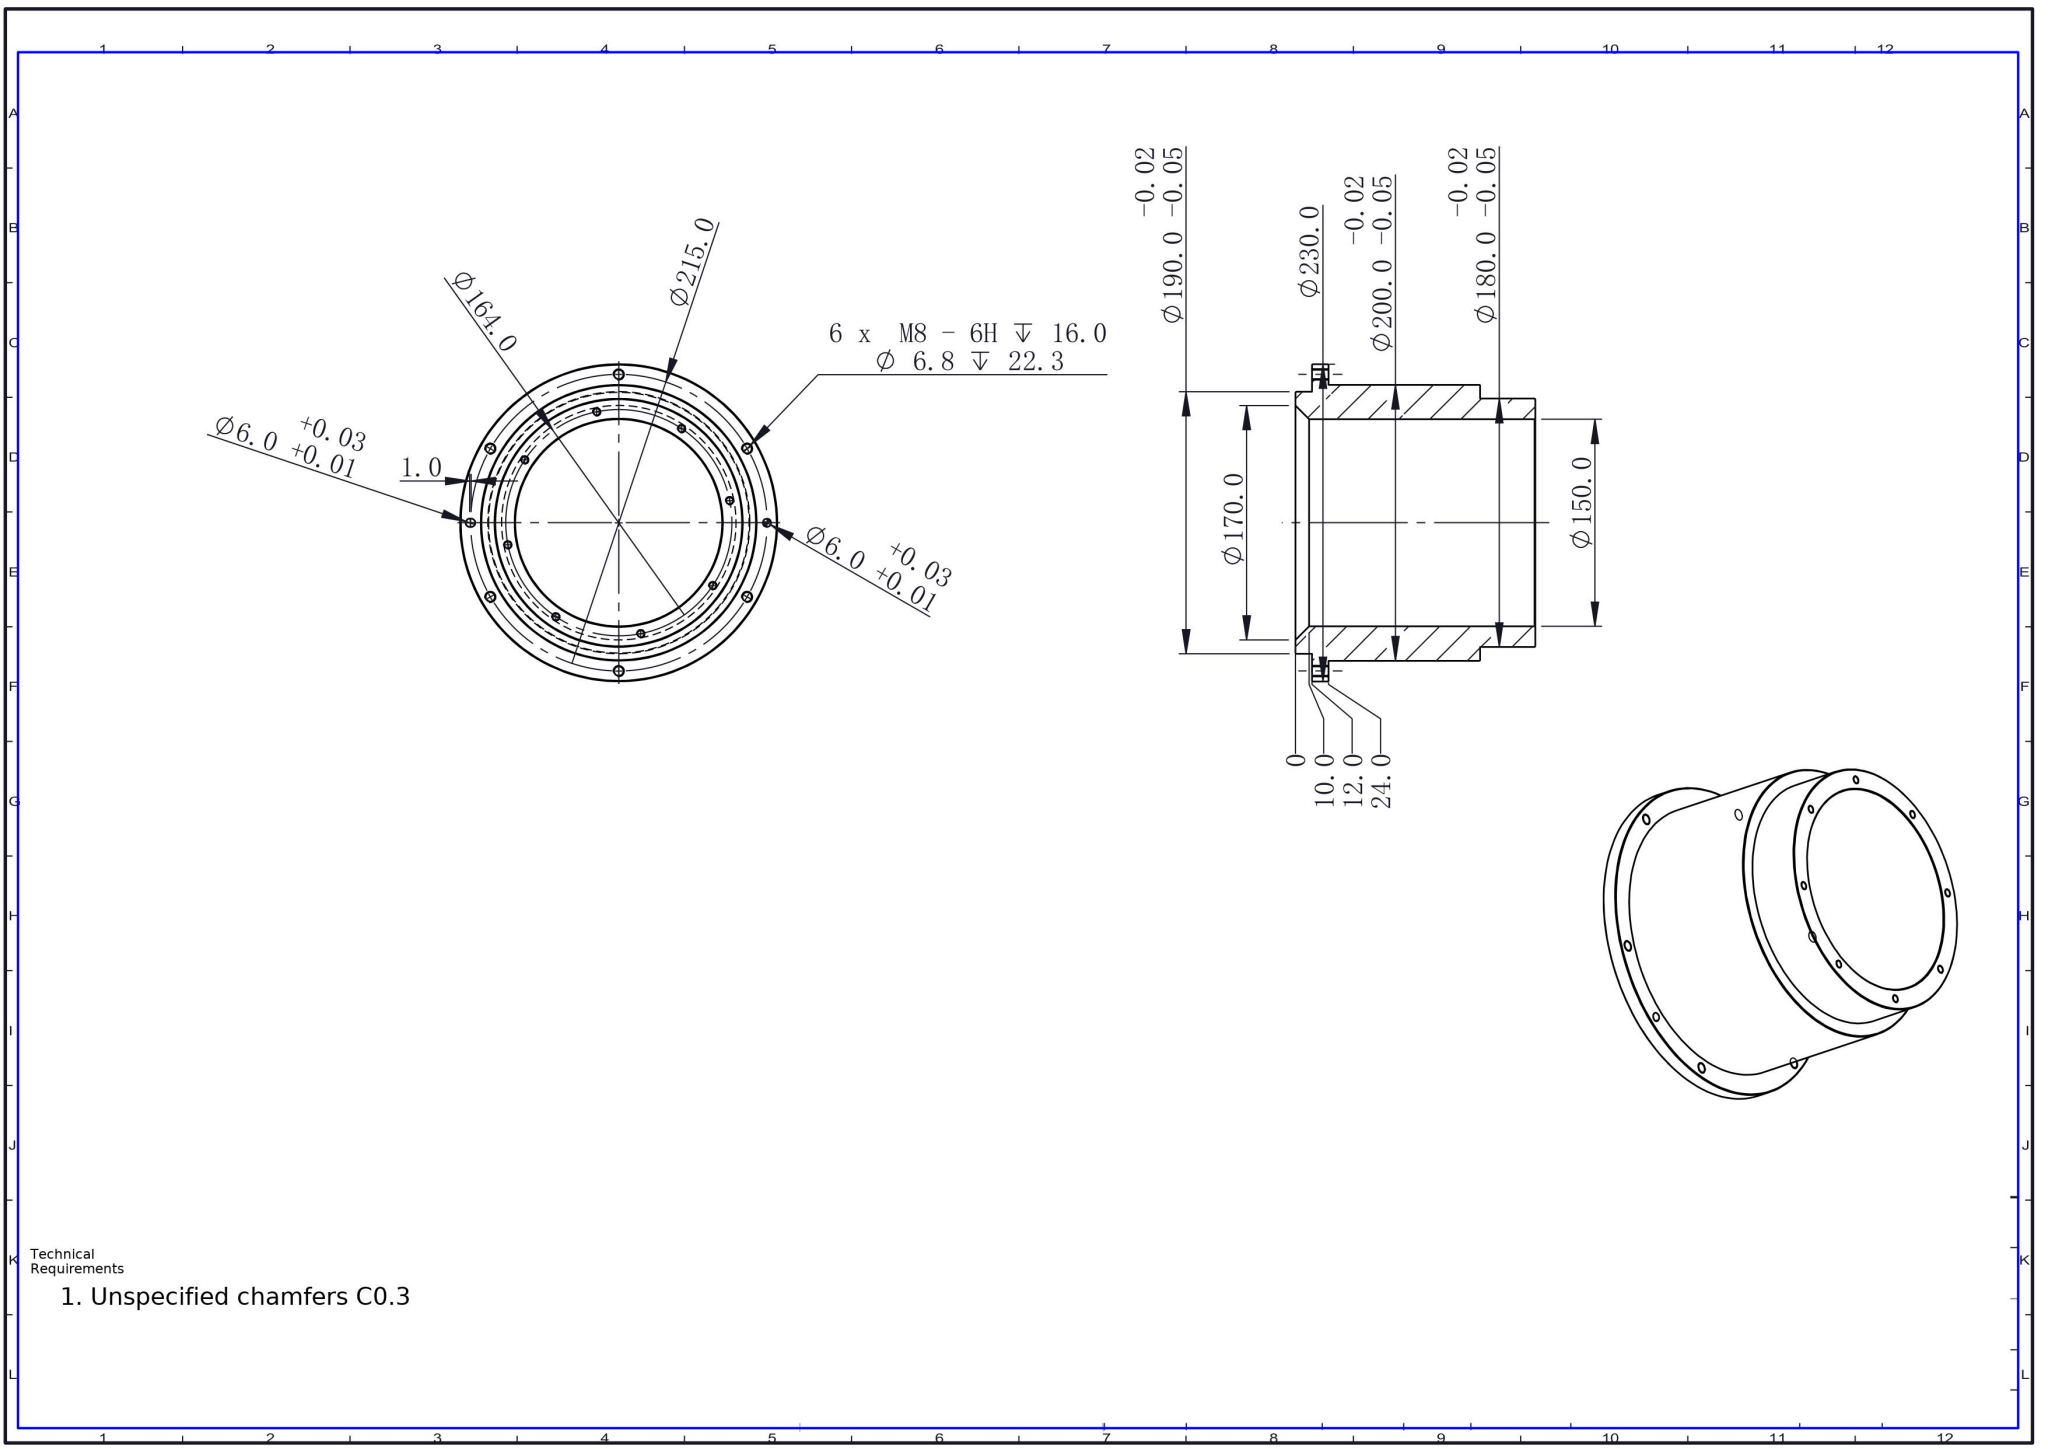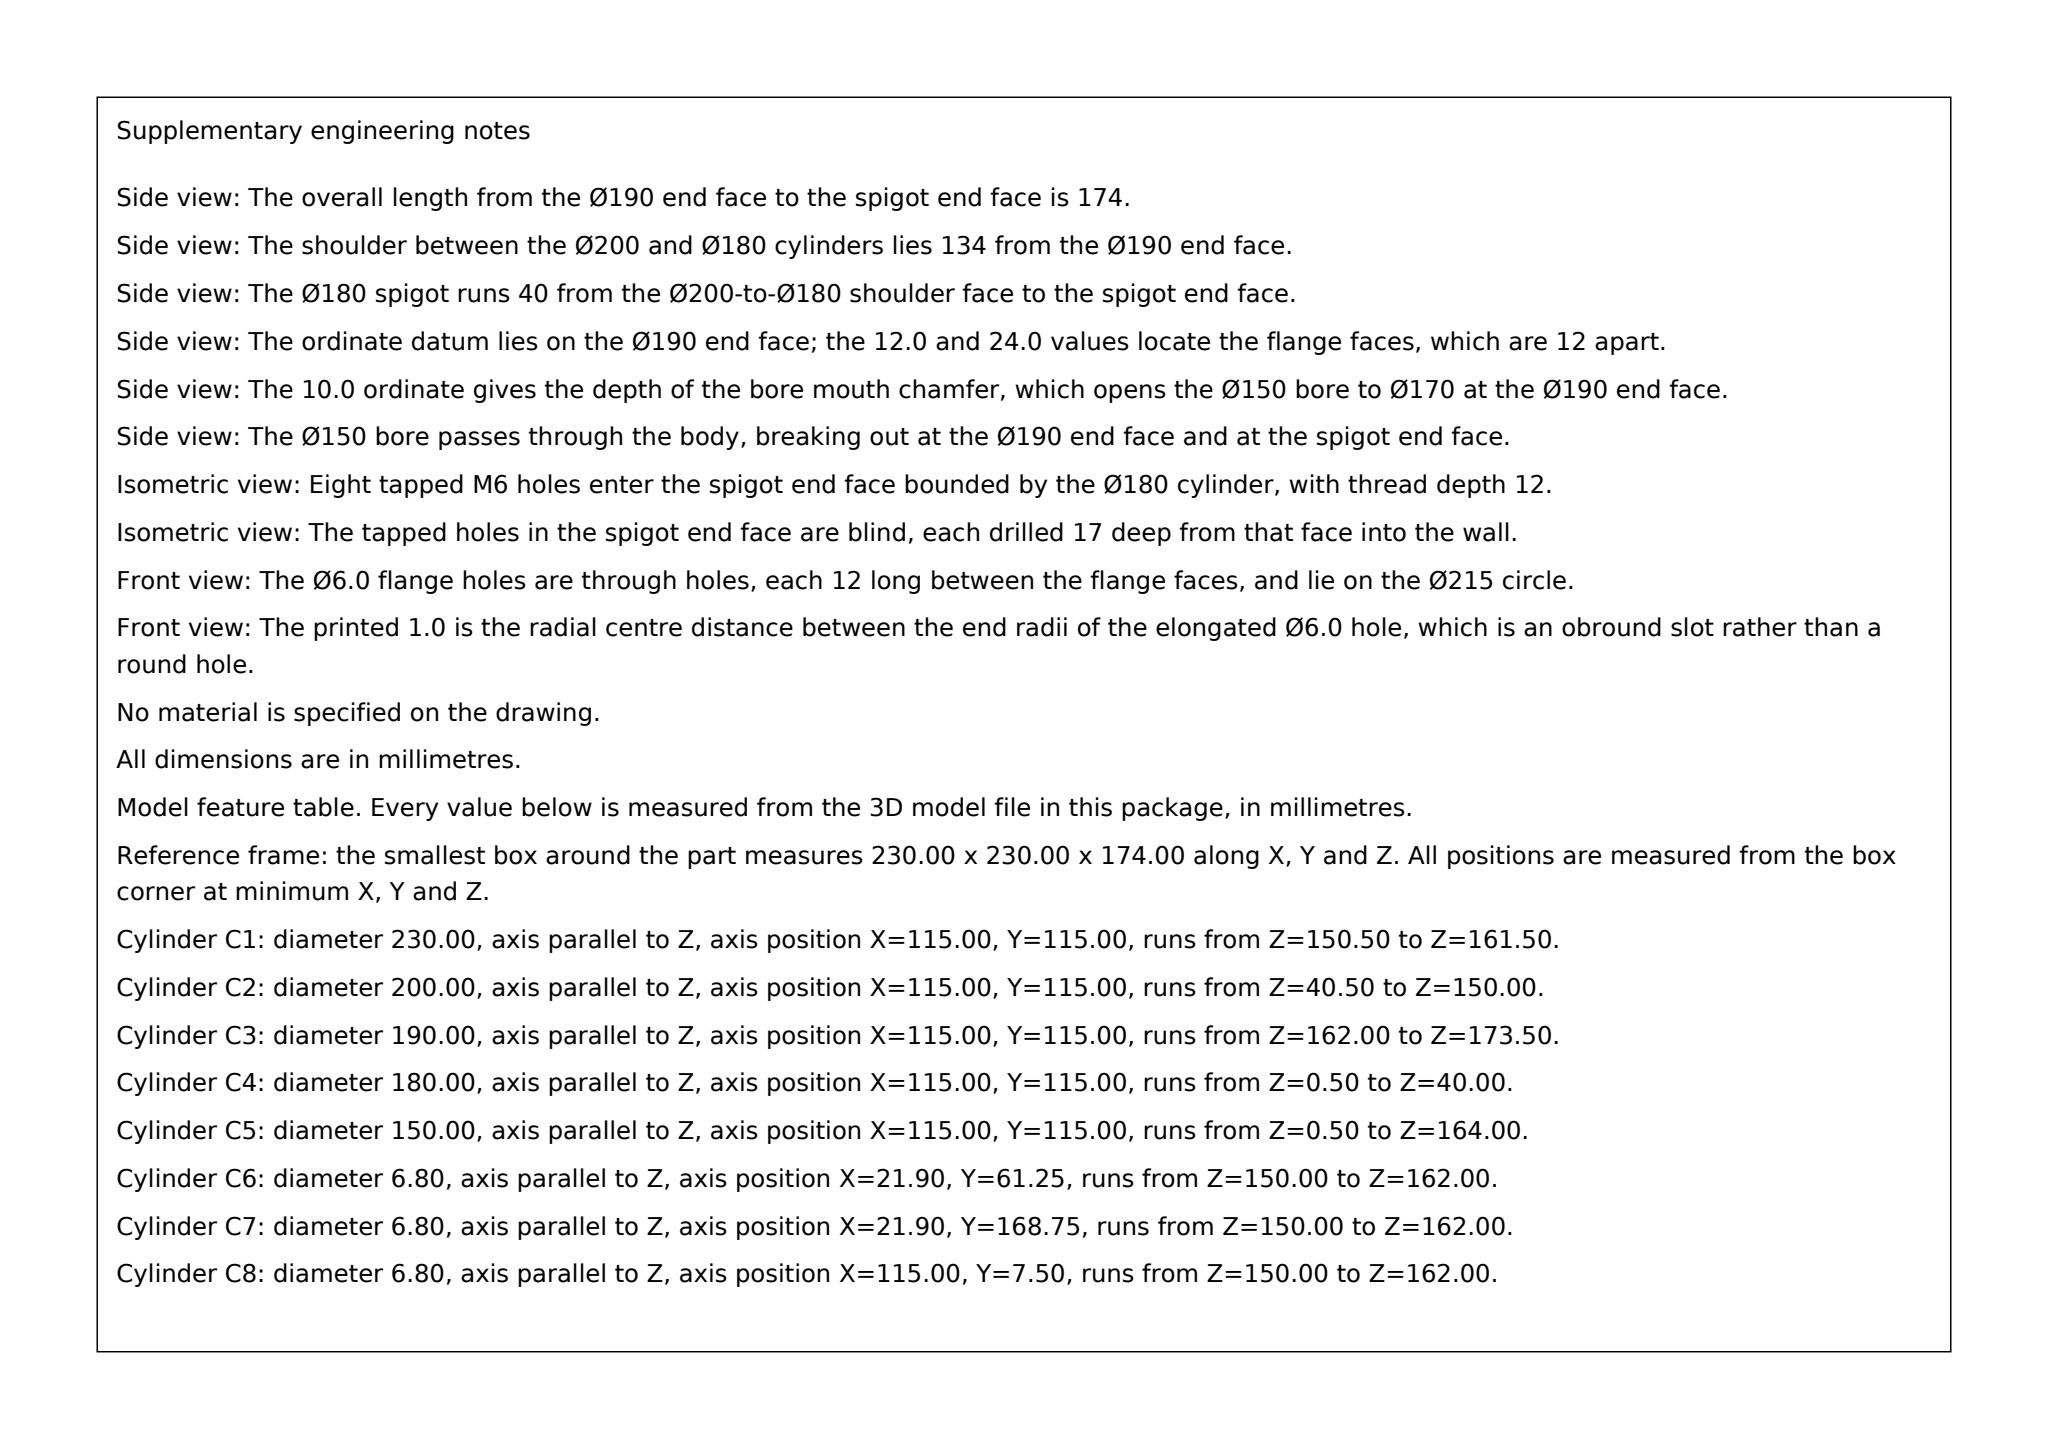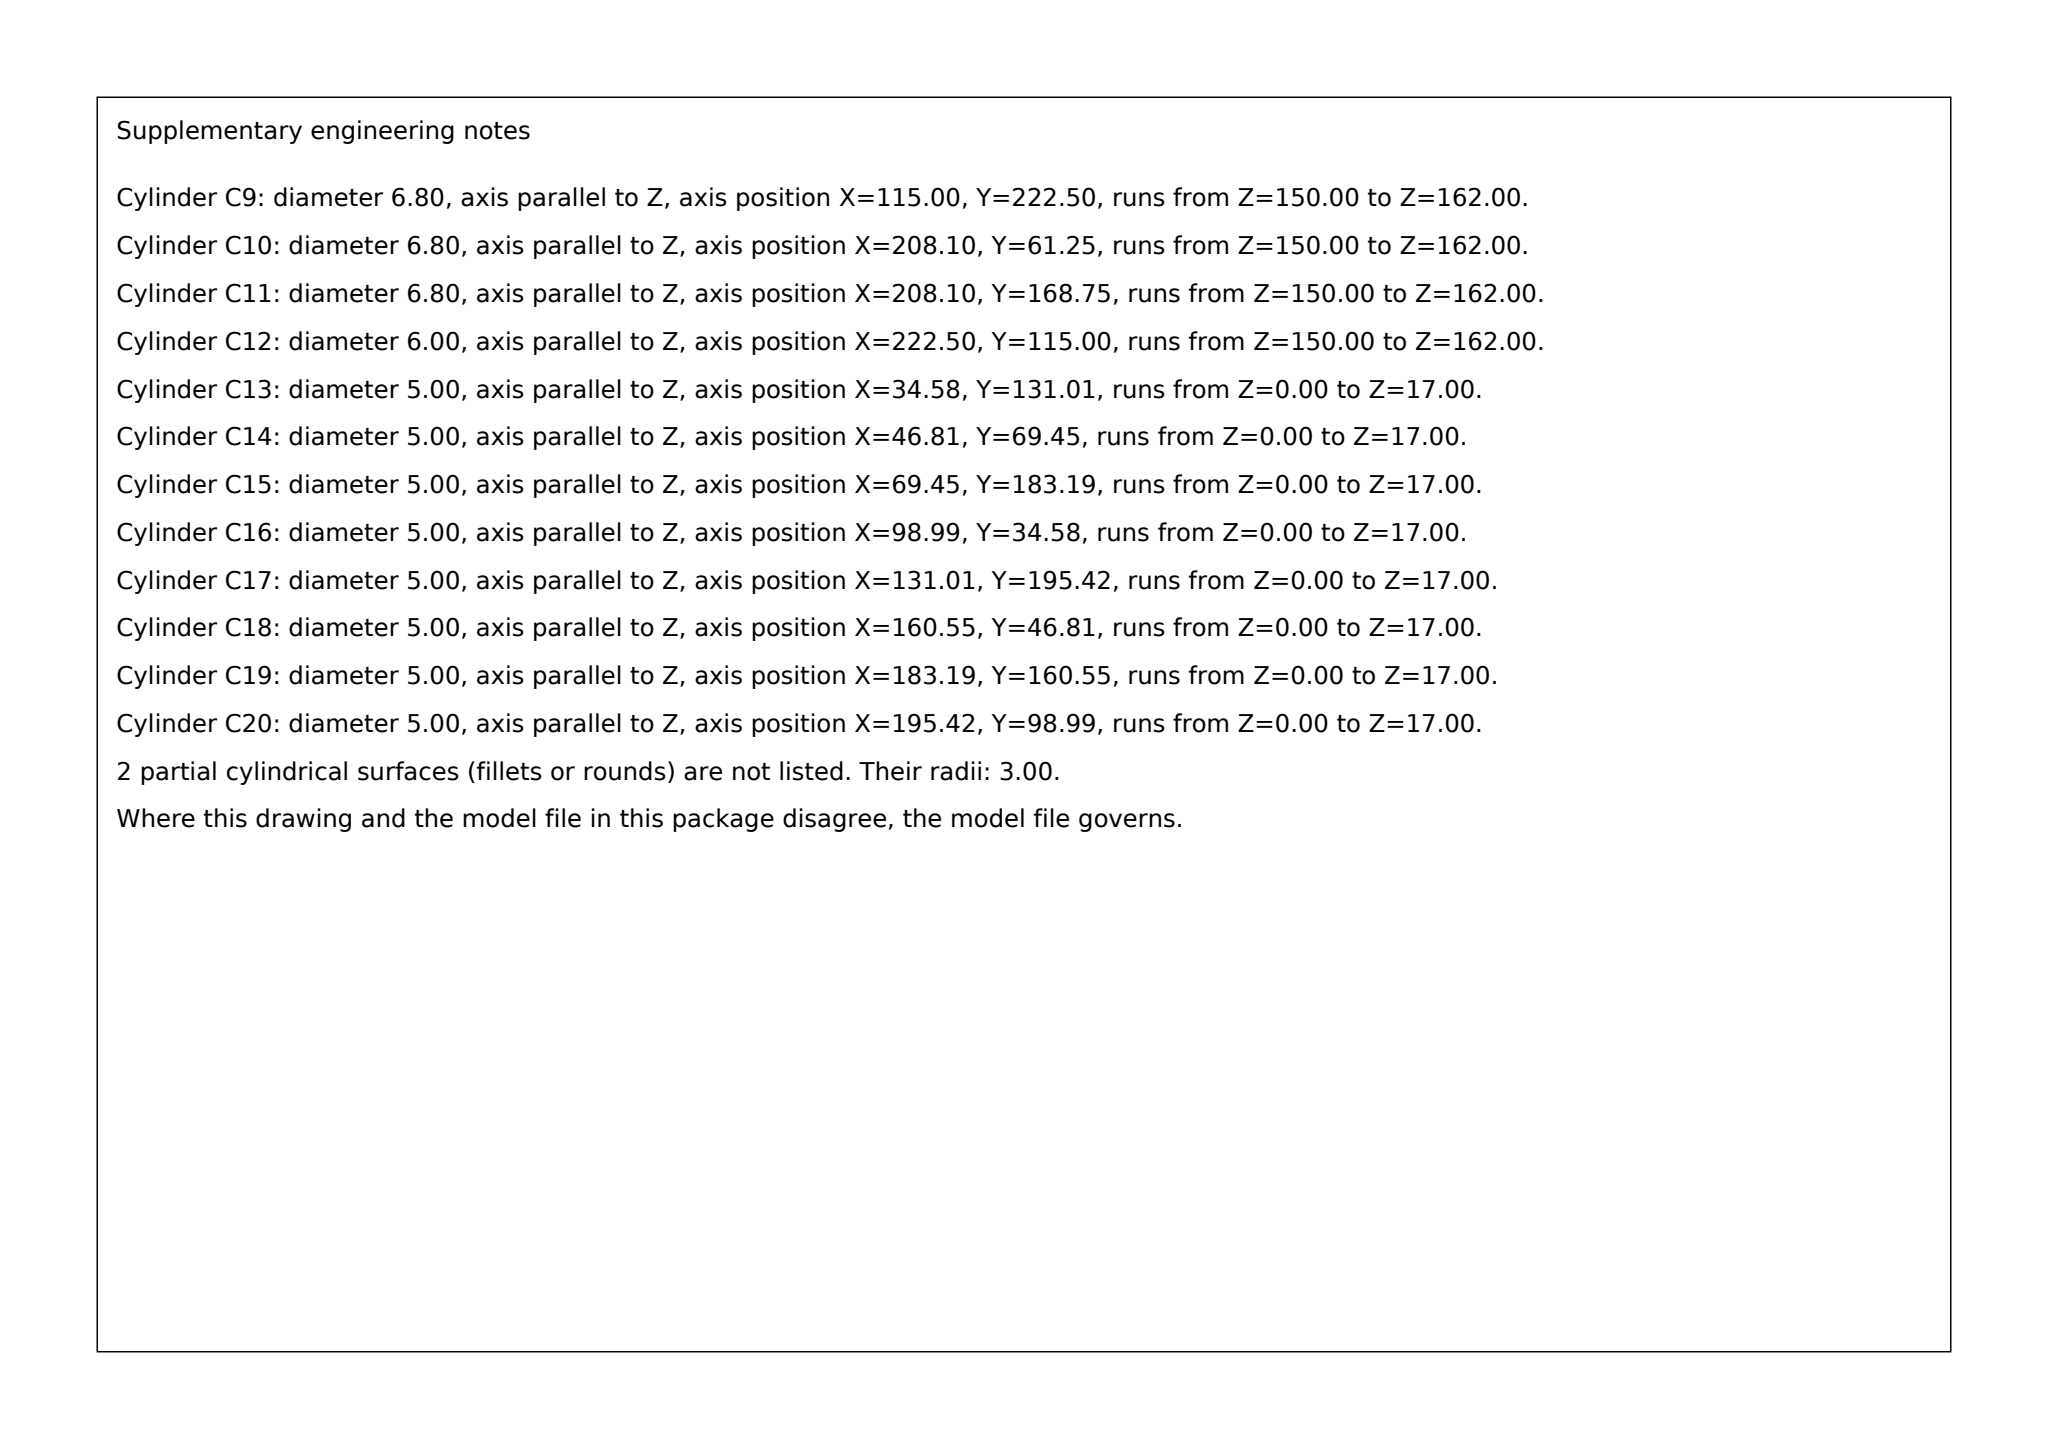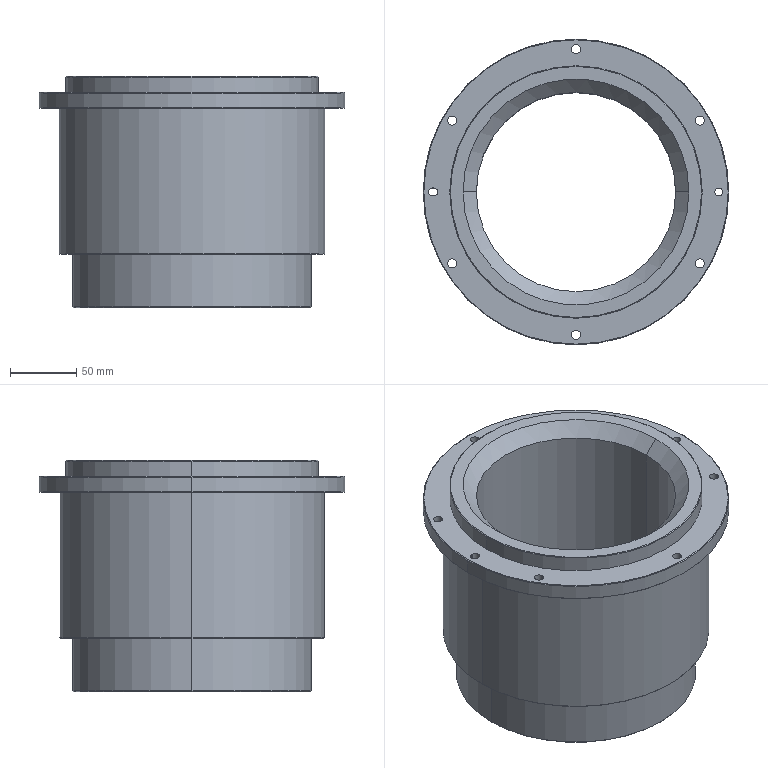Part | SolidWorks | mm | 1 solid | 80 faces | box 230 x 230 x 174 mm | volume 2206413 mm3 | cylinder 43 | cone 30 | plane 7 | commonest cylinder face diameters 5 x16 6.8 x12 6 x5 180 x2 200 x2 230 x2 190 x2 150 x2
Drawing notes:
6 x M8-6H EQL SP 60° ON Ø215 B.C., 1 HOLE ON VERT CL | from the solid: Ø6.8 holes at (21.9,61.25),(21.9,168.75),(115,7.5),(115,222.5),(208.1,61.25),(208.1,168.75); all R107.5 from axis (115,115) = Ø215 B.C., 60° spacing, one hole on vertical CL
2 x Ø6 +0.03/+0.01 ON Ø215 B.C., ON HORIZ CL, 180° APART | from the solid: Ø6 holes at (7.0/8.0,115) slot pair and (222.5,115); slot centre x=7.5, both y=115 (horiz CL), R107.5 from axis = Ø215 B.C.
2 x Ø6 +0.03/+0.01 DP 12.0 FROM FLANGE FACE (0 DATUM) | from the solid: Ø6.0 cylinders length 12.0, z from 0 face (z-planes 0, 40, 150, 162, 174)
C0.5 x 45° ON Ø230, Ø190, Ø200, Ø180 & Ø150 EDGES | from the solid: cones 90° incl between ref dia 230/229, 190/189, 200, 180, 151/150 = 0.5 x 45° chamfers
build123d program:
from build123d import *

# Parameters (mm, degrees)
CHAMFER1_SIZE                 = 10
M6_TAPPED_HOLE1_D             = 5
M6_TAPPED_HOLE1_DEPTH         = 17
M6_TAPPED_HOLE1_TIP           = 1.502
M8_TAPPED_HOLE1_D             = 6.8
M8_TAPPED_HOLE1_DEPTH         = 22.3
M8_TAPPED_HOLE1_TIP           = 2.043
SIZE_MM_DOWEL_PIN_HOLE1_D     = 6
SIZE_MM_DOWEL_PIN_HOLE1_DEPTH = 22.3
SIZE_MM_DOWEL_PIN_HOLE1_TIP   = 1.803
CUT_EXTRUDE1_DEPTH            = 55
CHAMFER2_SIZE                 = 0.5


with BuildPart() as part:
    # Sketch1 → Revolve1 (revolve)
    with BuildSketch(Plane(origin=(0, 0, 0), x_dir=(1, 0, 0), z_dir=(0, 1, 0)), mode=Mode.PRIVATE) as revolve1_sk:
        Polygon((-75, 0), (-95, 0), (-95, 12), (-115, 12), (-115, 24), (-100, 24), (-100, 134), (-90, 134), (-90, 174), (-75, 174), align=None)
    revolve(revolve1_sk.sketch.rotate(Axis((0, 0, 0), (0, 0, -1)), 180), axis=Axis((0, 0, 0), (0, 0, -1)))

    # Chamfer1
    chamfer1_edges = [part.edges().sort_by_distance(p)[0] for p in [
        (-75, 0, 0),
    ]]
    chamfer(chamfer1_edges, length=CHAMFER1_SIZE)

    # M6 Tapped Hole1
    with Locations(Plane(origin=(0, 0, -174), x_dir=(-1, 0, 0), z_dir=(0, 0, -1))):
        with Locations((-45.546, -68.188), (16.01, -80.422), (68.188, -45.546), (80.422, 16.01), (45.546, 68.188), (-16.01, 80.422), (-68.188, 45.546), (-80.422, -16.01)):
            Hole(M6_TAPPED_HOLE1_D / 2, depth=M6_TAPPED_HOLE1_DEPTH)
            with Locations((0, 0, -(M6_TAPPED_HOLE1_DEPTH + M6_TAPPED_HOLE1_TIP / 2))):  # 118° drill point
                Cone(0, M6_TAPPED_HOLE1_D / 2, M6_TAPPED_HOLE1_TIP, mode=Mode.SUBTRACT)

    # M8 Tapped Hole1
    with Locations(Plane(origin=(0, 0, -24), x_dir=(-1, 0, 0), z_dir=(0, 0, -1))):
        with Locations((-93.098, 53.75), (0, 107.5), (93.098, 53.75), (93.098, -53.75), (0, -107.5), (-93.098, -53.75)):
            Hole(M8_TAPPED_HOLE1_D / 2, depth=M8_TAPPED_HOLE1_DEPTH)
            with Locations((0, 0, -(M8_TAPPED_HOLE1_DEPTH + M8_TAPPED_HOLE1_TIP / 2))):  # 118° drill point
                Cone(0, M8_TAPPED_HOLE1_D / 2, M8_TAPPED_HOLE1_TIP, mode=Mode.SUBTRACT)

    # Size mm Dowel Pin Hole1
    with Locations(Plane(origin=(0, 0, -24), x_dir=(-1, 0, 0), z_dir=(0, 0, -1))):
        with Locations((-107.5, 0)):
            Hole(SIZE_MM_DOWEL_PIN_HOLE1_D / 2, depth=SIZE_MM_DOWEL_PIN_HOLE1_DEPTH)
            with Locations((0, 0, -(SIZE_MM_DOWEL_PIN_HOLE1_DEPTH + SIZE_MM_DOWEL_PIN_HOLE1_TIP / 2))):  # 118° drill point
                Cone(0, SIZE_MM_DOWEL_PIN_HOLE1_D / 2, SIZE_MM_DOWEL_PIN_HOLE1_TIP, mode=Mode.SUBTRACT)

    # Sketch12 → Cut-Extrude1 (cut)
    with BuildSketch(Plane(origin=(0, 0, -24), x_dir=(-1, 0, 0), z_dir=(0, 0, -1))):
        with BuildLine():
            Line((107, 3), (108, 3))
            ThreePointArc((108, 3), (111, 0), (108, -3))
            Line((108, -3), (107, -3))
            ThreePointArc((107, -3), (104, 0), (107, 3))
        make_face()
    extrude(amount=-CUT_EXTRUDE1_DEPTH, mode=Mode.SUBTRACT)

    # Chamfer2
    chamfer2_edges = [part.edges().sort_by_distance(p)[0] for p in [
        (-115, 0, -24),
        (-115, 0, -12),
        (-95, 0, 0),
        (-75, 0, -174),
        (-90, 0, -174),
        (-100, 0, -134),
    ]]
    chamfer(chamfer2_edges, length=CHAMFER2_SIZE)


solid = part.part